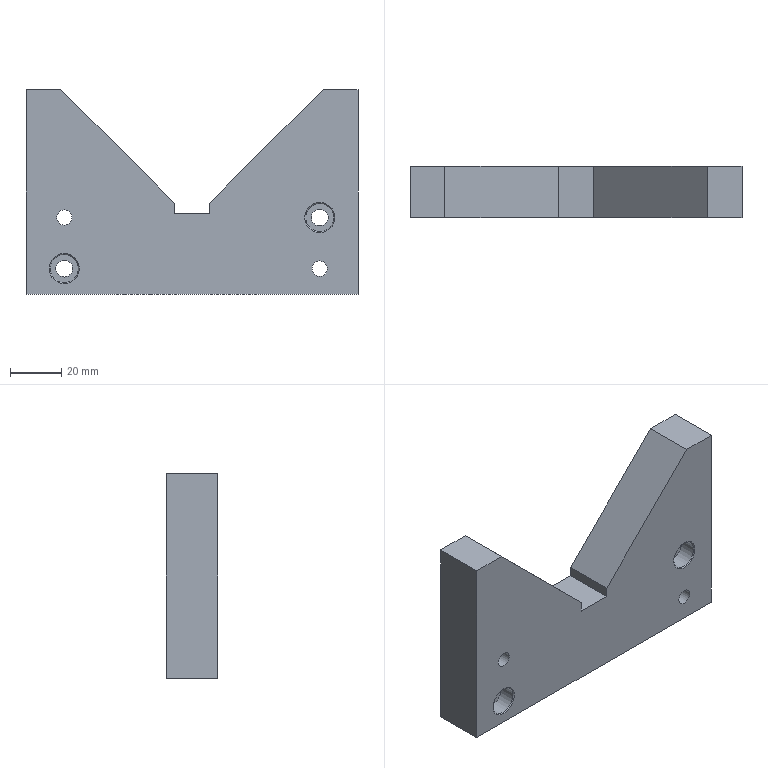Component | NX | FIXED_V_BLOCK | 1 solid | 24 faces | volume 151855 mm3 | plane 14 | cylinder 6 | cone 4 | commonest cylinder face diameters 6.6 x2 11 x2 6 x2